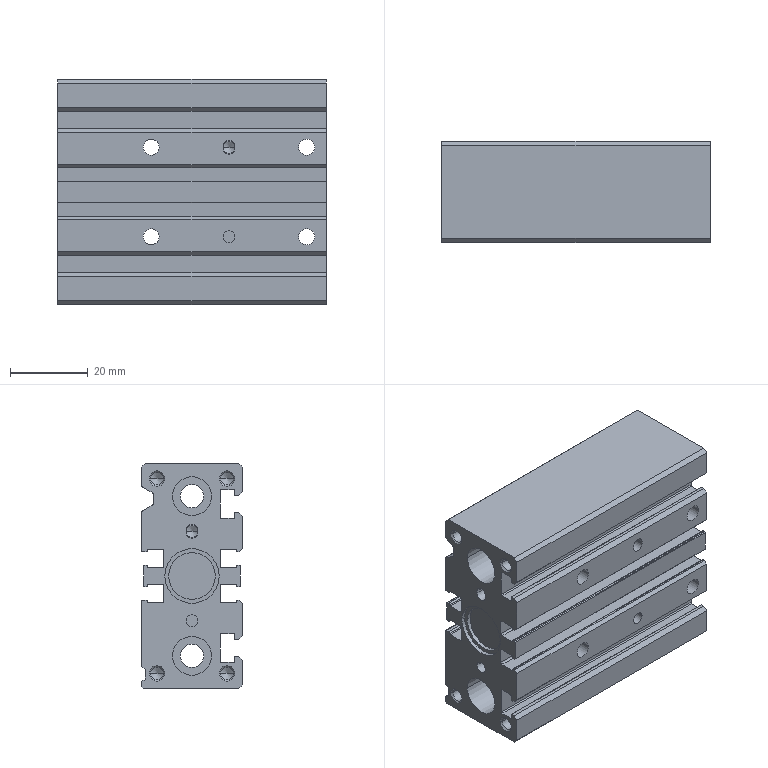Component | SolidWorks | Inline-H010-TCL12x40S_0_+_CS1-G-1-3_Inline-H010-TCL12x40SCylinder-1 | 1 solid | 279 faces | volume 74405 mm3 | cylinder 124 | plane 101 | cone 52 | spline 2 | commonest cylinder face diameters 0.8 x20 3 x12 4.134 x12 0.4 x12 12 x10 3.242 x8 8 x8 4.3 x8